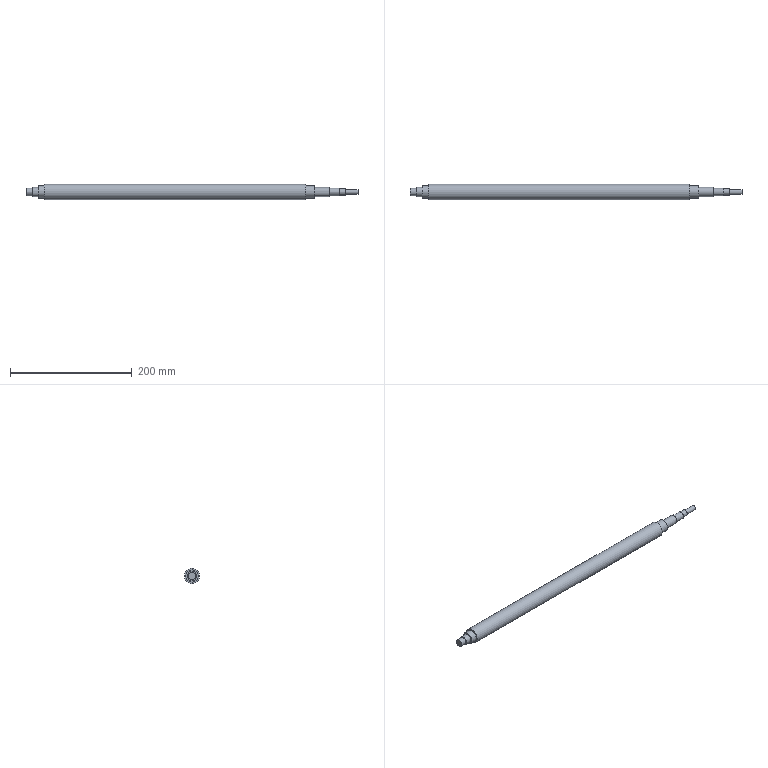Component | NX | X_LEADSCREW | 1 solid | 19 faces | box 546 x 25 x 25 mm | volume 229782 mm3 | plane 10 | cylinder 9 | commonest cylinder face diameters 12 x2 15 x2 20 x2 8 x1 10 x1 25 x1
STEP:
#1=CARTESIAN_POINT('',(0.,0.,0.));
#2=DIRECTION('',(0.,0.,1.));
#3=DIRECTION('',(1.,0.,0.));
#4=AXIS2_PLACEMENT_3D('',#1,#2,#3);
#5=CARTESIAN_POINT('',(417.689,-150.302,-1579.));
#6=VERTEX_POINT('',#5);
#7=CARTESIAN_POINT('',(417.689,-150.302,-1573.));
#8=DIRECTION('',(1.,0.,0.));
#9=DIRECTION('',(0.,0.,-1.));
#10=AXIS2_PLACEMENT_3D('',#7,#8,#9);
#11=CIRCLE('',#10,6.);
#12=CARTESIAN_POINT('',(417.689,-150.302,-1573.));
#13=DIRECTION('',(1.,0.,0.));
#14=DIRECTION('',(0.,0.,-1.));
#15=AXIS2_PLACEMENT_3D('',#12,#13,#14);
#16=PLANE('',#15);
#17=CARTESIAN_POINT('',(0.,0.));
#18=DIRECTION('',(1.,0.));
#19=AXIS2_PLACEMENT_2D('',#17,#18);
#20=CIRCLE('',#19,6.);
#21=(GEOMETRIC_REPRESENTATION_CONTEXT(2)PARAMETRIC_REPRESENTATION_CONTEXT()REPRESENTATION_CONTEXT('',''));
#22=DEFINITIONAL_REPRESENTATION('',(#20),#21);
#23=PCURVE('',#16,#22);
#24=CARTESIAN_POINT('',(662.689,-150.302,-1573.));
#25=DIRECTION('',(1.,0.,0.));
#26=DIRECTION('',(0.,0.,-1.));
#27=AXIS2_PLACEMENT_3D('',#24,#25,#26);
#28=CYLINDRICAL_SURFACE('',#27,6.);
#29=CARTESIAN_POINT('',(0.,-245.));
#30=DIRECTION('',(1.,0.));
#31=VECTOR('',#30,1.);
#32=LINE('',#29,#31);
#33=(GEOMETRIC_REPRESENTATION_CONTEXT(2)PARAMETRIC_REPRESENTATION_CONTEXT()REPRESENTATION_CONTEXT('',''));
#34=DEFINITIONAL_REPRESENTATION('',(#32),#33);
#35=PCURVE('',#28,#34);
#36=SURFACE_CURVE('',#11,(#23,#35),.PCURVE_S1.);
#37=EDGE_CURVE('',#6,#6,#36,.T.);
#38=ORIENTED_EDGE('',*,*,#37,.F.);
#39=EDGE_LOOP('',(#38));
#40=FACE_BOUND('',#39,.T.);
#41=ADVANCED_FACE('',(#40),#16,.F.);
#42=CARTESIAN_POINT('',(963.689,-150.302,-1577.));
#43=VERTEX_POINT('',#42);
#44=CARTESIAN_POINT('',(963.689,-150.302,-1573.));
#45=DIRECTION('',(1.,0.,0.));
#46=DIRECTION('',(0.,0.,-1.));
#47=AXIS2_PLACEMENT_3D('',#44,#45,#46);
#48=CIRCLE('',#47,4.);
#49=CARTESIAN_POINT('',(963.689,-150.302,-1573.));
#50=DIRECTION('',(1.,0.,0.));
#51=DIRECTION('',(0.,0.,-1.));
#52=AXIS2_PLACEMENT_3D('',#49,#50,#51);
#53=PLANE('',#52);
#54=CARTESIAN_POINT('',(0.,0.));
#55=DIRECTION('',(1.,0.));
#56=AXIS2_PLACEMENT_2D('',#54,#55);
#57=CIRCLE('',#56,4.);
#58=(GEOMETRIC_REPRESENTATION_CONTEXT(2)PARAMETRIC_REPRESENTATION_CONTEXT()REPRESENTATION_CONTEXT('',''));
#59=DEFINITIONAL_REPRESENTATION('',(#57),#58);
#60=PCURVE('',#53,#59);
#61=CARTESIAN_POINT('',(662.689,-150.302,-1573.));
#62=DIRECTION('',(1.,0.,0.));
#63=DIRECTION('',(0.,0.,-1.));
#64=AXIS2_PLACEMENT_3D('',#61,#62,#63);
#65=CYLINDRICAL_SURFACE('',#64,4.);
#66=CARTESIAN_POINT('',(0.,301.));
#67=DIRECTION('',(1.,0.));
#68=VECTOR('',#67,1.);
#69=LINE('',#66,#68);
#70=(GEOMETRIC_REPRESENTATION_CONTEXT(2)PARAMETRIC_REPRESENTATION_CONTEXT()REPRESENTATION_CONTEXT('',''));
#71=DEFINITIONAL_REPRESENTATION('',(#69),#70);
#72=PCURVE('',#65,#71);
#73=SURFACE_CURVE('',#48,(#60,#72),.PCURVE_S1.);
#74=EDGE_CURVE('',#43,#43,#73,.T.);
#75=ORIENTED_EDGE('',*,*,#74,.T.);
#76=EDGE_LOOP('',(#75));
#77=FACE_BOUND('',#76,.T.);
#78=ADVANCED_FACE('',(#77),#53,.T.);
#79=ORIENTED_EDGE('',*,*,#74,.F.);
#80=CARTESIAN_POINT('',(943.689,-150.302,-1577.));
#81=VERTEX_POINT('',#80);
#82=CARTESIAN_POINT('',(943.689,-150.302,-1577.));
#83=CARTESIAN_POINT('',(963.689,-150.302,-1577.));
#84=B_SPLINE_CURVE_WITH_KNOTS('',1,(#82,#83),.UNSPECIFIED.,.F.,.F.,(2,2),(281.,301.),.PIECEWISE_BEZIER_KNOTS.);
#85=CARTESIAN_POINT('',(0.,0.));
#86=DIRECTION('',(0.,1.));
#87=VECTOR('',#86,1.);
#88=LINE('',#85,#87);
#89=(GEOMETRIC_REPRESENTATION_CONTEXT(2)PARAMETRIC_REPRESENTATION_CONTEXT()REPRESENTATION_CONTEXT('',''));
#90=DEFINITIONAL_REPRESENTATION('',(#88),#89);
#91=PCURVE('',#65,#90);
#92=CARTESIAN_POINT('',(6.283,0.));
#93=DIRECTION('',(0.,1.));
#94=VECTOR('',#93,1.);
#95=LINE('',#92,#94);
#96=(GEOMETRIC_REPRESENTATION_CONTEXT(2)PARAMETRIC_REPRESENTATION_CONTEXT()REPRESENTATION_CONTEXT('',''));
#97=DEFINITIONAL_REPRESENTATION('',(#95),#96);
#98=PCURVE('',#65,#97);
#99=SEAM_CURVE('',#84,(#91,#98),.PCURVE_S1.);
#100=EDGE_CURVE('',#81,#43,#99,.T.);
#101=ORIENTED_EDGE('',*,*,#100,.F.);
#102=CARTESIAN_POINT('',(943.689,-150.302,-1573.));
#103=DIRECTION('',(1.,0.,0.));
#104=DIRECTION('',(0.,0.,-1.));
#105=AXIS2_PLACEMENT_3D('',#102,#103,#104);
#106=CIRCLE('',#105,4.);
#107=CARTESIAN_POINT('',(0.,281.));
#108=DIRECTION('',(1.,0.));
#109=VECTOR('',#108,1.);
#110=LINE('',#107,#109);
#111=(GEOMETRIC_REPRESENTATION_CONTEXT(2)PARAMETRIC_REPRESENTATION_CONTEXT()REPRESENTATION_CONTEXT('',''));
#112=DEFINITIONAL_REPRESENTATION('',(#110),#111);
#113=PCURVE('',#65,#112);
#114=CARTESIAN_POINT('',(943.689,-150.302,-1568.));
#115=DIRECTION('',(-1.,0.,0.));
#116=DIRECTION('',(0.,0.,1.));
#117=AXIS2_PLACEMENT_3D('',#114,#115,#116);
#118=PLANE('',#117);
#119=CARTESIAN_POINT('',(-9.,0.));
#120=CARTESIAN_POINT('',(-9.,6.928));
#121=CARTESIAN_POINT('',(-3.,3.464));
#122=CARTESIAN_POINT('',(3.,0.));
#123=CARTESIAN_POINT('',(-3.,-3.464));
#124=CARTESIAN_POINT('',(-9.,-6.928));
#125=CARTESIAN_POINT('',(-9.,0.));
#126=(BOUNDED_CURVE()B_SPLINE_CURVE(2,(#119,#120,#121,#122,#123,#124,#125),.UNSPECIFIED.,.T.,.F.)B_SPLINE_CURVE_WITH_KNOTS((1,2,2,2,2,1),(-2.094,0.,2.094,4.189,6.283,8.378),.UNSPECIFIED.)CURVE()GEOMETRIC_REPRESENTATION_ITEM()RATIONAL_B_SPLINE_CURVE((1.,0.5,1.,0.5,1.,0.5,1.))REPRESENTATION_ITEM(''));
#127=(GEOMETRIC_REPRESENTATION_CONTEXT(2)PARAMETRIC_REPRESENTATION_CONTEXT()REPRESENTATION_CONTEXT('',''));
#128=DEFINITIONAL_REPRESENTATION('',(#126),#127);
#129=PCURVE('',#118,#128);
#130=SURFACE_CURVE('',#106,(#113,#129),.PCURVE_S1.);
#131=EDGE_CURVE('',#81,#81,#130,.T.);
#132=ORIENTED_EDGE('',*,*,#131,.T.);
#133=ORIENTED_EDGE('',*,*,#100,.T.);
#134=EDGE_LOOP('',(#79,#101,#132,#133));
#135=FACE_BOUND('',#134,.T.);
#136=ADVANCED_FACE('',(#135),#65,.T.);
#137=ORIENTED_EDGE('',*,*,#131,.F.);
#138=EDGE_LOOP('',(#137));
#139=FACE_BOUND('',#138,.T.);
#140=CARTESIAN_POINT('',(943.689,-150.302,-1578.));
#141=VERTEX_POINT('',#140);
#142=CARTESIAN_POINT('',(943.689,-150.302,-1573.));
#143=DIRECTION('',(1.,0.,0.));
#144=DIRECTION('',(0.,0.,-1.));
#145=AXIS2_PLACEMENT_3D('',#142,#143,#144);
#146=CIRCLE('',#145,5.);
#147=CARTESIAN_POINT('',(-10.,0.));
#148=CARTESIAN_POINT('',(-10.,8.66));
#149=CARTESIAN_POINT('',(-2.5,4.33));
#150=CARTESIAN_POINT('',(5.,0.));
#151=CARTESIAN_POINT('',(-2.5,-4.33));
#152=CARTESIAN_POINT('',(-10.,-8.66));
#153=CARTESIAN_POINT('',(-10.,0.));
#154=(BOUNDED_CURVE()B_SPLINE_CURVE(2,(#147,#148,#149,#150,#151,#152,#153),.UNSPECIFIED.,.T.,.F.)B_SPLINE_CURVE_WITH_KNOTS((1,2,2,2,2,1),(-2.094,0.,2.094,4.189,6.283,8.378),.UNSPECIFIED.)CURVE()GEOMETRIC_REPRESENTATION_ITEM()RATIONAL_B_SPLINE_CURVE((1.,0.5,1.,0.5,1.,0.5,1.))REPRESENTATION_ITEM(''));
#155=(GEOMETRIC_REPRESENTATION_CONTEXT(2)PARAMETRIC_REPRESENTATION_CONTEXT()REPRESENTATION_CONTEXT('',''));
#156=DEFINITIONAL_REPRESENTATION('',(#154),#155);
#157=PCURVE('',#118,#156);
#158=CARTESIAN_POINT('',(662.689,-150.302,-1573.));
#159=DIRECTION('',(1.,0.,0.));
#160=DIRECTION('',(0.,0.,-1.));
#161=AXIS2_PLACEMENT_3D('',#158,#159,#160);
#162=CYLINDRICAL_SURFACE('',#161,5.);
#163=CARTESIAN_POINT('',(0.,281.));
#164=DIRECTION('',(1.,0.));
#165=VECTOR('',#164,1.);
#166=LINE('',#163,#165);
#167=(GEOMETRIC_REPRESENTATION_CONTEXT(2)PARAMETRIC_REPRESENTATION_CONTEXT()REPRESENTATION_CONTEXT('',''));
#168=DEFINITIONAL_REPRESENTATION('',(#166),#167);
#169=PCURVE('',#162,#168);
#170=SURFACE_CURVE('',#146,(#157,#169),.PCURVE_S1.);
#171=EDGE_CURVE('',#141,#141,#170,.T.);
#172=ORIENTED_EDGE('',*,*,#171,.T.);
#173=EDGE_LOOP('',(#172));
#174=FACE_BOUND('',#173,.T.);
#175=ADVANCED_FACE('',(#139,#174),#118,.F.);
#176=ORIENTED_EDGE('',*,*,#171,.F.);
#177=CARTESIAN_POINT('',(933.689,-150.302,-1578.));
#178=VERTEX_POINT('',#177);
#179=CARTESIAN_POINT('',(933.689,-150.302,-1578.));
#180=CARTESIAN_POINT('',(943.689,-150.302,-1578.));
#181=B_SPLINE_CURVE_WITH_KNOTS('',1,(#179,#180),.UNSPECIFIED.,.F.,.F.,(2,2),(271.,281.),.PIECEWISE_BEZIER_KNOTS.);
#182=CARTESIAN_POINT('',(0.,0.));
#183=DIRECTION('',(0.,1.));
#184=VECTOR('',#183,1.);
#185=LINE('',#182,#184);
#186=(GEOMETRIC_REPRESENTATION_CONTEXT(2)PARAMETRIC_REPRESENTATION_CONTEXT()REPRESENTATION_CONTEXT('',''));
#187=DEFINITIONAL_REPRESENTATION('',(#185),#186);
#188=PCURVE('',#162,#187);
#189=CARTESIAN_POINT('',(6.283,0.));
#190=DIRECTION('',(0.,1.));
#191=VECTOR('',#190,1.);
#192=LINE('',#189,#191);
#193=(GEOMETRIC_REPRESENTATION_CONTEXT(2)PARAMETRIC_REPRESENTATION_CONTEXT()REPRESENTATION_CONTEXT('',''));
#194=DEFINITIONAL_REPRESENTATION('',(#192),#193);
#195=PCURVE('',#162,#194);
#196=SEAM_CURVE('',#181,(#188,#195),.PCURVE_S1.);
#197=EDGE_CURVE('',#178,#141,#196,.T.);
#198=ORIENTED_EDGE('',*,*,#197,.F.);
#199=CARTESIAN_POINT('',(933.689,-150.302,-1573.));
#200=DIRECTION('',(1.,0.,0.));
#201=DIRECTION('',(0.,0.,-1.));
#202=AXIS2_PLACEMENT_3D('',#199,#200,#201);
#203=CIRCLE('',#202,5.);
#204=CARTESIAN_POINT('',(0.,271.));
#205=DIRECTION('',(1.,0.));
#206=VECTOR('',#205,1.);
#207=LINE('',#204,#206);
#208=(GEOMETRIC_REPRESENTATION_CONTEXT(2)PARAMETRIC_REPRESENTATION_CONTEXT()REPRESENTATION_CONTEXT('',''));
#209=DEFINITIONAL_REPRESENTATION('',(#207),#208);
#210=PCURVE('',#162,#209);
#211=CARTESIAN_POINT('',(933.689,-150.302,-1567.));
#212=DIRECTION('',(-1.,0.,0.));
#213=DIRECTION('',(0.,0.,1.));
#214=AXIS2_PLACEMENT_3D('',#211,#212,#213);
#215=PLANE('',#214);
#216=CARTESIAN_POINT('',(-11.,0.));
#217=CARTESIAN_POINT('',(-11.,8.66));
#218=CARTESIAN_POINT('',(-3.5,4.33));
#219=CARTESIAN_POINT('',(4.,0.));
#220=CARTESIAN_POINT('',(-3.5,-4.33));
#221=CARTESIAN_POINT('',(-11.,-8.66));
#222=CARTESIAN_POINT('',(-11.,0.));
#223=(BOUNDED_CURVE()B_SPLINE_CURVE(2,(#216,#217,#218,#219,#220,#221,#222),.UNSPECIFIED.,.T.,.F.)B_SPLINE_CURVE_WITH_KNOTS((1,2,2,2,2,1),(-2.094,0.,2.094,4.189,6.283,8.378),.UNSPECIFIED.)CURVE()GEOMETRIC_REPRESENTATION_ITEM()RATIONAL_B_SPLINE_CURVE((1.,0.5,1.,0.5,1.,0.5,1.))REPRESENTATION_ITEM(''));
#224=(GEOMETRIC_REPRESENTATION_CONTEXT(2)PARAMETRIC_REPRESENTATION_CONTEXT()REPRESENTATION_CONTEXT('',''));
#225=DEFINITIONAL_REPRESENTATION('',(#223),#224);
#226=PCURVE('',#215,#225);
#227=SURFACE_CURVE('',#203,(#210,#226),.PCURVE_S1.);
#228=EDGE_CURVE('',#178,#178,#227,.T.);
#229=ORIENTED_EDGE('',*,*,#228,.T.);
#230=ORIENTED_EDGE('',*,*,#197,.T.);
#231=EDGE_LOOP('',(#176,#198,#229,#230));
#232=FACE_BOUND('',#231,.T.);
#233=ADVANCED_FACE('',(#232),#162,.T.);
#234=ORIENTED_EDGE('',*,*,#228,.F.);
#235=EDGE_LOOP('',(#234));
#236=FACE_BOUND('',#235,.T.);
#237=CARTESIAN_POINT('',(933.689,-150.302,-1579.));
#238=VERTEX_POINT('',#237);
#239=CARTESIAN_POINT('',(933.689,-150.302,-1573.));
#240=DIRECTION('',(1.,0.,0.));
#241=DIRECTION('',(0.,0.,-1.));
#242=AXIS2_PLACEMENT_3D('',#239,#240,#241);
#243=CIRCLE('',#242,6.);
#244=CARTESIAN_POINT('',(-12.,0.));
#245=CARTESIAN_POINT('',(-12.,10.392));
#246=CARTESIAN_POINT('',(-3.,5.196));
#247=CARTESIAN_POINT('',(6.,0.));
#248=CARTESIAN_POINT('',(-3.,-5.196));
#249=CARTESIAN_POINT('',(-12.,-10.392));
#250=CARTESIAN_POINT('',(-12.,0.));
#251=(BOUNDED_CURVE()B_SPLINE_CURVE(2,(#244,#245,#246,#247,#248,#249,#250),.UNSPECIFIED.,.T.,.F.)B_SPLINE_CURVE_WITH_KNOTS((1,2,2,2,2,1),(-2.094,0.,2.094,4.189,6.283,8.378),.UNSPECIFIED.)CURVE()GEOMETRIC_REPRESENTATION_ITEM()RATIONAL_B_SPLINE_CURVE((1.,0.5,1.,0.5,1.,0.5,1.))REPRESENTATION_ITEM(''));
#252=(GEOMETRIC_REPRESENTATION_CONTEXT(2)PARAMETRIC_REPRESENTATION_CONTEXT()REPRESENTATION_CONTEXT('',''));
#253=DEFINITIONAL_REPRESENTATION('',(#251),#252);
#254=PCURVE('',#215,#253);
#255=CARTESIAN_POINT('',(662.689,-150.302,-1573.));
#256=DIRECTION('',(1.,0.,0.));
#257=DIRECTION('',(0.,0.,-1.));
#258=AXIS2_PLACEMENT_3D('',#255,#256,#257);
#259=CYLINDRICAL_SURFACE('',#258,6.);
#260=CARTESIAN_POINT('',(0.,271.));
#261=DIRECTION('',(1.,0.));
#262=VECTOR('',#261,1.);
#263=LINE('',#260,#262);
#264=(GEOMETRIC_REPRESENTATION_CONTEXT(2)PARAMETRIC_REPRESENTATION_CONTEXT()REPRESENTATION_CONTEXT('',''));
#265=DEFINITIONAL_REPRESENTATION('',(#263),#264);
#266=PCURVE('',#259,#265);
#267=SURFACE_CURVE('',#243,(#254,#266),.PCURVE_S1.);
#268=EDGE_CURVE('',#238,#238,#267,.T.);
#269=ORIENTED_EDGE('',*,*,#268,.T.);
#270=EDGE_LOOP('',(#269));
#271=FACE_BOUND('',#270,.T.);
#272=ADVANCED_FACE('',(#236,#271),#215,.F.);
#273=ORIENTED_EDGE('',*,*,#268,.F.);
#274=CARTESIAN_POINT('',(916.689,-150.302,-1579.));
#275=VERTEX_POINT('',#274);
#276=CARTESIAN_POINT('',(916.689,-150.302,-1579.));
#277=CARTESIAN_POINT('',(933.689,-150.302,-1579.));
#278=B_SPLINE_CURVE_WITH_KNOTS('',1,(#276,#277),.UNSPECIFIED.,.F.,.F.,(2,2),(254.,271.),.PIECEWISE_BEZIER_KNOTS.);
#279=CARTESIAN_POINT('',(0.,0.));
#280=DIRECTION('',(0.,1.));
#281=VECTOR('',#280,1.);
#282=LINE('',#279,#281);
#283=(GEOMETRIC_REPRESENTATION_CONTEXT(2)PARAMETRIC_REPRESENTATION_CONTEXT()REPRESENTATION_CONTEXT('',''));
#284=DEFINITIONAL_REPRESENTATION('',(#282),#283);
#285=PCURVE('',#259,#284);
#286=CARTESIAN_POINT('',(6.283,0.));
#287=DIRECTION('',(0.,1.));
#288=VECTOR('',#287,1.);
#289=LINE('',#286,#288);
#290=(GEOMETRIC_REPRESENTATION_CONTEXT(2)PARAMETRIC_REPRESENTATION_CONTEXT()REPRESENTATION_CONTEXT('',''));
#291=DEFINITIONAL_REPRESENTATION('',(#289),#290);
#292=PCURVE('',#259,#291);
#293=SEAM_CURVE('',#278,(#285,#292),.PCURVE_S1.);
#294=EDGE_CURVE('',#275,#238,#293,.T.);
#295=ORIENTED_EDGE('',*,*,#294,.F.);
#296=CARTESIAN_POINT('',(916.689,-150.302,-1573.));
#297=DIRECTION('',(1.,0.,0.));
#298=DIRECTION('',(0.,0.,-1.));
#299=AXIS2_PLACEMENT_3D('',#296,#297,#298);
#300=CIRCLE('',#299,6.);
#301=CARTESIAN_POINT('',(0.,254.));
#302=DIRECTION('',(1.,0.));
#303=VECTOR('',#302,1.);
#304=LINE('',#301,#303);
#305=(GEOMETRIC_REPRESENTATION_CONTEXT(2)PARAMETRIC_REPRESENTATION_CONTEXT()REPRESENTATION_CONTEXT('',''));
#306=DEFINITIONAL_REPRESENTATION('',(#304),#305);
#307=PCURVE('',#259,#306);
#308=CARTESIAN_POINT('',(916.689,-150.302,-1565.5));
#309=DIRECTION('',(-1.,0.,0.));
#310=DIRECTION('',(0.,0.,1.));
#311=AXIS2_PLACEMENT_3D('',#308,#309,#310);
#312=PLANE('',#311);
#313=CARTESIAN_POINT('',(-13.5,0.));
#314=CARTESIAN_POINT('',(-13.5,10.392));
#315=CARTESIAN_POINT('',(-4.5,5.196));
#316=CARTESIAN_POINT('',(4.5,0.));
#317=CARTESIAN_POINT('',(-4.5,-5.196));
#318=CARTESIAN_POINT('',(-13.5,-10.392));
#319=CARTESIAN_POINT('',(-13.5,0.));
#320=(BOUNDED_CURVE()B_SPLINE_CURVE(2,(#313,#314,#315,#316,#317,#318,#319),.UNSPECIFIED.,.T.,.F.)B_SPLINE_CURVE_WITH_KNOTS((1,2,2,2,2,1),(-2.094,0.,2.094,4.189,6.283,8.378),.UNSPECIFIED.)CURVE()GEOMETRIC_REPRESENTATION_ITEM()RATIONAL_B_SPLINE_CURVE((1.,0.5,1.,0.5,1.,0.5,1.))REPRESENTATION_ITEM(''));
#321=(GEOMETRIC_REPRESENTATION_CONTEXT(2)PARAMETRIC_REPRESENTATION_CONTEXT()REPRESENTATION_CONTEXT('',''));
#322=DEFINITIONAL_REPRESENTATION('',(#320),#321);
#323=PCURVE('',#312,#322);
#324=SURFACE_CURVE('',#300,(#307,#323),.PCURVE_S1.);
#325=EDGE_CURVE('',#275,#275,#324,.T.);
#326=ORIENTED_EDGE('',*,*,#325,.T.);
#327=ORIENTED_EDGE('',*,*,#294,.T.);
#328=EDGE_LOOP('',(#273,#295,#326,#327));
#329=FACE_BOUND('',#328,.T.);
#330=ADVANCED_FACE('',(#329),#259,.T.);
#331=ORIENTED_EDGE('',*,*,#325,.F.);
#332=EDGE_LOOP('',(#331));
#333=FACE_BOUND('',#332,.T.);
#334=CARTESIAN_POINT('',(916.689,-150.302,-1580.5));
#335=VERTEX_POINT('',#334);
#336=CARTESIAN_POINT('',(916.689,-150.302,-1573.));
#337=DIRECTION('',(1.,0.,0.));
#338=DIRECTION('',(0.,0.,-1.));
#339=AXIS2_PLACEMENT_3D('',#336,#337,#338);
#340=CIRCLE('',#339,7.5);
#341=CARTESIAN_POINT('',(-15.,0.));
#342=CARTESIAN_POINT('',(-15.,12.99));
#343=CARTESIAN_POINT('',(-3.75,6.495));
#344=CARTESIAN_POINT('',(7.5,0.));
#345=CARTESIAN_POINT('',(-3.75,-6.495));
#346=CARTESIAN_POINT('',(-15.,-12.99));
#347=CARTESIAN_POINT('',(-15.,0.));
#348=(BOUNDED_CURVE()B_SPLINE_CURVE(2,(#341,#342,#343,#344,#345,#346,#347),.UNSPECIFIED.,.T.,.F.)B_SPLINE_CURVE_WITH_KNOTS((1,2,2,2,2,1),(-2.094,0.,2.094,4.189,6.283,8.378),.UNSPECIFIED.)CURVE()GEOMETRIC_REPRESENTATION_ITEM()RATIONAL_B_SPLINE_CURVE((1.,0.5,1.,0.5,1.,0.5,1.))REPRESENTATION_ITEM(''));
#349=(GEOMETRIC_REPRESENTATION_CONTEXT(2)PARAMETRIC_REPRESENTATION_CONTEXT()REPRESENTATION_CONTEXT('',''));
#350=DEFINITIONAL_REPRESENTATION('',(#348),#349);
#351=PCURVE('',#312,#350);
#352=CARTESIAN_POINT('',(662.689,-150.302,-1573.));
#353=DIRECTION('',(1.,0.,0.));
#354=DIRECTION('',(0.,0.,-1.));
#355=AXIS2_PLACEMENT_3D('',#352,#353,#354);
#356=CYLINDRICAL_SURFACE('',#355,7.5);
#357=CARTESIAN_POINT('',(0.,254.));
#358=DIRECTION('',(1.,0.));
#359=VECTOR('',#358,1.);
#360=LINE('',#357,#359);
#361=(GEOMETRIC_REPRESENTATION_CONTEXT(2)PARAMETRIC_REPRESENTATION_CONTEXT()REPRESENTATION_CONTEXT('',''));
#362=DEFINITIONAL_REPRESENTATION('',(#360),#361);
#363=PCURVE('',#356,#362);
#364=SURFACE_CURVE('',#340,(#351,#363),.PCURVE_S1.);
#365=EDGE_CURVE('',#335,#335,#364,.T.);
#366=ORIENTED_EDGE('',*,*,#365,.T.);
#367=EDGE_LOOP('',(#366));
#368=FACE_BOUND('',#367,.T.);
#369=ADVANCED_FACE('',(#333,#368),#312,.F.);
#370=ORIENTED_EDGE('',*,*,#365,.F.);
#371=CARTESIAN_POINT('',(892.689,-150.302,-1580.5));
#372=VERTEX_POINT('',#371);
#373=CARTESIAN_POINT('',(892.689,-150.302,-1580.5));
#374=CARTESIAN_POINT('',(916.689,-150.302,-1580.5));
#375=B_SPLINE_CURVE_WITH_KNOTS('',1,(#373,#374),.UNSPECIFIED.,.F.,.F.,(2,2),(230.,254.),.PIECEWISE_BEZIER_KNOTS.);
#376=CARTESIAN_POINT('',(0.,0.));
#377=DIRECTION('',(0.,1.));
#378=VECTOR('',#377,1.);
#379=LINE('',#376,#378);
#380=(GEOMETRIC_REPRESENTATION_CONTEXT(2)PARAMETRIC_REPRESENTATION_CONTEXT()REPRESENTATION_CONTEXT('',''));
#381=DEFINITIONAL_REPRESENTATION('',(#379),#380);
#382=PCURVE('',#356,#381);
#383=CARTESIAN_POINT('',(6.283,0.));
#384=DIRECTION('',(0.,1.));
#385=VECTOR('',#384,1.);
#386=LINE('',#383,#385);
#387=(GEOMETRIC_REPRESENTATION_CONTEXT(2)PARAMETRIC_REPRESENTATION_CONTEXT()REPRESENTATION_CONTEXT('',''));
#388=DEFINITIONAL_REPRESENTATION('',(#386),#387);
#389=PCURVE('',#356,#388);
#390=SEAM_CURVE('',#375,(#382,#389),.PCURVE_S1.);
#391=EDGE_CURVE('',#372,#335,#390,.T.);
#392=ORIENTED_EDGE('',*,*,#391,.F.);
#393=CARTESIAN_POINT('',(892.689,-150.302,-1573.));
#394=DIRECTION('',(1.,0.,0.));
#395=DIRECTION('',(0.,0.,-1.));
#396=AXIS2_PLACEMENT_3D('',#393,#394,#395);
#397=CIRCLE('',#396,7.5);
#398=CARTESIAN_POINT('',(0.,230.));
#399=DIRECTION('',(1.,0.));
#400=VECTOR('',#399,1.);
#401=LINE('',#398,#400);
#402=(GEOMETRIC_REPRESENTATION_CONTEXT(2)PARAMETRIC_REPRESENTATION_CONTEXT()REPRESENTATION_CONTEXT('',''));
#403=DEFINITIONAL_REPRESENTATION('',(#401),#402);
#404=PCURVE('',#356,#403);
#405=CARTESIAN_POINT('',(892.689,-150.302,-1563.));
#406=DIRECTION('',(-1.,0.,0.));
#407=DIRECTION('',(0.,0.,1.));
#408=AXIS2_PLACEMENT_3D('',#405,#406,#407);
#409=PLANE('',#408);
#410=CARTESIAN_POINT('',(-17.5,0.));
#411=CARTESIAN_POINT('',(-17.5,12.99));
#412=CARTESIAN_POINT('',(-6.25,6.495));
#413=CARTESIAN_POINT('',(5.,0.));
#414=CARTESIAN_POINT('',(-6.25,-6.495));
#415=CARTESIAN_POINT('',(-17.5,-12.99));
#416=CARTESIAN_POINT('',(-17.5,0.));
#417=(BOUNDED_CURVE()B_SPLINE_CURVE(2,(#410,#411,#412,#413,#414,#415,#416),.UNSPECIFIED.,.T.,.F.)B_SPLINE_CURVE_WITH_KNOTS((1,2,2,2,2,1),(-2.094,0.,2.094,4.189,6.283,8.378),.UNSPECIFIED.)CURVE()GEOMETRIC_REPRESENTATION_ITEM()RATIONAL_B_SPLINE_CURVE((1.,0.5,1.,0.5,1.,0.5,1.))REPRESENTATION_ITEM(''));
#418=(GEOMETRIC_REPRESENTATION_CONTEXT(2)PARAMETRIC_REPRESENTATION_CONTEXT()REPRESENTATION_CONTEXT('',''));
#419=DEFINITIONAL_REPRESENTATION('',(#417),#418);
#420=PCURVE('',#409,#419);
#421=SURFACE_CURVE('',#397,(#404,#420),.PCURVE_S1.);
#422=EDGE_CURVE('',#372,#372,#421,.T.);
#423=ORIENTED_EDGE('',*,*,#422,.T.);
#424=ORIENTED_EDGE('',*,*,#391,.T.);
#425=EDGE_LOOP('',(#370,#392,#423,#424));
#426=FACE_BOUND('',#425,.T.);
#427=ADVANCED_FACE('',(#426),#356,.T.);
#428=ORIENTED_EDGE('',*,*,#422,.F.);
#429=EDGE_LOOP('',(#428));
#430=FACE_BOUND('',#429,.T.);
#431=CARTESIAN_POINT('',(892.689,-150.302,-1583.));
#432=VERTEX_POINT('',#431);
#433=CARTESIAN_POINT('',(892.689,-150.302,-1573.));
#434=DIRECTION('',(1.,0.,0.));
#435=DIRECTION('',(0.,0.,-1.));
#436=AXIS2_PLACEMENT_3D('',#433,#434,#435);
#437=CIRCLE('',#436,10.);
#438=CARTESIAN_POINT('',(-20.,0.));
#439=CARTESIAN_POINT('',(-20.,17.321));
#440=CARTESIAN_POINT('',(-5.,8.66));
#441=CARTESIAN_POINT('',(10.,0.));
#442=CARTESIAN_POINT('',(-5.,-8.66));
#443=CARTESIAN_POINT('',(-20.,-17.321));
#444=CARTESIAN_POINT('',(-20.,0.));
#445=(BOUNDED_CURVE()B_SPLINE_CURVE(2,(#438,#439,#440,#441,#442,#443,#444),.UNSPECIFIED.,.T.,.F.)B_SPLINE_CURVE_WITH_KNOTS((1,2,2,2,2,1),(-2.094,0.,2.094,4.189,6.283,8.378),.UNSPECIFIED.)CURVE()GEOMETRIC_REPRESENTATION_ITEM()RATIONAL_B_SPLINE_CURVE((1.,0.5,1.,0.5,1.,0.5,1.))REPRESENTATION_ITEM(''));
#446=(GEOMETRIC_REPRESENTATION_CONTEXT(2)PARAMETRIC_REPRESENTATION_CONTEXT()REPRESENTATION_CONTEXT('',''));
#447=DEFINITIONAL_REPRESENTATION('',(#445),#446);
#448=PCURVE('',#409,#447);
#449=CARTESIAN_POINT('',(662.689,-150.302,-1573.));
#450=DIRECTION('',(1.,0.,0.));
#451=DIRECTION('',(0.,0.,-1.));
#452=AXIS2_PLACEMENT_3D('',#449,#450,#451);
#453=CYLINDRICAL_SURFACE('',#452,10.);
#454=CARTESIAN_POINT('',(0.,230.));
#455=DIRECTION('',(1.,0.));
#456=VECTOR('',#455,1.);
#457=LINE('',#454,#456);
#458=(GEOMETRIC_REPRESENTATION_CONTEXT(2)PARAMETRIC_REPRESENTATION_CONTEXT()REPRESENTATION_CONTEXT('',''));
#459=DEFINITIONAL_REPRESENTATION('',(#457),#458);
#460=PCURVE('',#453,#459);
#461=SURFACE_CURVE('',#437,(#448,#460),.PCURVE_S1.);
#462=EDGE_CURVE('',#432,#432,#461,.T.);
#463=ORIENTED_EDGE('',*,*,#462,.T.);
#464=EDGE_LOOP('',(#463));
#465=FACE_BOUND('',#464,.T.);
#466=ADVANCED_FACE('',(#430,#465),#409,.F.);
#467=ORIENTED_EDGE('',*,*,#462,.F.);
#468=CARTESIAN_POINT('',(877.689,-150.302,-1583.));
#469=VERTEX_POINT('',#468);
#470=CARTESIAN_POINT('',(877.689,-150.302,-1583.));
#471=CARTESIAN_POINT('',(892.689,-150.302,-1583.));
#472=B_SPLINE_CURVE_WITH_KNOTS('',1,(#470,#471),.UNSPECIFIED.,.F.,.F.,(2,2),(215.,230.),.PIECEWISE_BEZIER_KNOTS.);
#473=CARTESIAN_POINT('',(0.,0.));
#474=DIRECTION('',(0.,1.));
#475=VECTOR('',#474,1.);
#476=LINE('',#473,#475);
#477=(GEOMETRIC_REPRESENTATION_CONTEXT(2)PARAMETRIC_REPRESENTATION_CONTEXT()REPRESENTATION_CONTEXT('',''));
#478=DEFINITIONAL_REPRESENTATION('',(#476),#477);
#479=PCURVE('',#453,#478);
#480=CARTESIAN_POINT('',(6.283,0.));
#481=DIRECTION('',(0.,1.));
#482=VECTOR('',#481,1.);
#483=LINE('',#480,#482);
#484=(GEOMETRIC_REPRESENTATION_CONTEXT(2)PARAMETRIC_REPRESENTATION_CONTEXT()REPRESENTATION_CONTEXT('',''));
#485=DEFINITIONAL_REPRESENTATION('',(#483),#484);
#486=PCURVE('',#453,#485);
#487=SEAM_CURVE('',#472,(#479,#486),.PCURVE_S1.);
#488=EDGE_CURVE('',#469,#432,#487,.T.);
#489=ORIENTED_EDGE('',*,*,#488,.F.);
#490=CARTESIAN_POINT('',(877.689,-150.302,-1573.));
#491=DIRECTION('',(1.,0.,0.));
#492=DIRECTION('',(0.,0.,-1.));
#493=AXIS2_PLACEMENT_3D('',#490,#491,#492);
#494=CIRCLE('',#493,10.);
#495=CARTESIAN_POINT('',(0.,215.));
#496=DIRECTION('',(1.,0.));
#497=VECTOR('',#496,1.);
#498=LINE('',#495,#497);
#499=(GEOMETRIC_REPRESENTATION_CONTEXT(2)PARAMETRIC_REPRESENTATION_CONTEXT()REPRESENTATION_CONTEXT('',''));
#500=DEFINITIONAL_REPRESENTATION('',(#498),#499);
#501=PCURVE('',#453,#500);
#502=CARTESIAN_POINT('',(877.689,-150.302,-1560.5));
#503=DIRECTION('',(-1.,0.,0.));
#504=DIRECTION('',(0.,0.,1.));
#505=AXIS2_PLACEMENT_3D('',#502,#503,#504);
#506=PLANE('',#505);
#507=CARTESIAN_POINT('',(-22.5,0.));
#508=CARTESIAN_POINT('',(-22.5,17.321));
#509=CARTESIAN_POINT('',(-7.5,8.66));
#510=CARTESIAN_POINT('',(7.5,0.));
#511=CARTESIAN_POINT('',(-7.5,-8.66));
#512=CARTESIAN_POINT('',(-22.5,-17.321));
#513=CARTESIAN_POINT('',(-22.5,0.));
#514=(BOUNDED_CURVE()B_SPLINE_CURVE(2,(#507,#508,#509,#510,#511,#512,#513),.UNSPECIFIED.,.T.,.F.)B_SPLINE_CURVE_WITH_KNOTS((1,2,2,2,2,1),(-2.094,0.,2.094,4.189,6.283,8.378),.UNSPECIFIED.)CURVE()GEOMETRIC_REPRESENTATION_ITEM()RATIONAL_B_SPLINE_CURVE((1.,0.5,1.,0.5,1.,0.5,1.))REPRESENTATION_ITEM(''));
#515=(GEOMETRIC_REPRESENTATION_CONTEXT(2)PARAMETRIC_REPRESENTATION_CONTEXT()REPRESENTATION_CONTEXT('',''));
#516=DEFINITIONAL_REPRESENTATION('',(#514),#515);
#517=PCURVE('',#506,#516);
#518=SURFACE_CURVE('',#494,(#501,#517),.PCURVE_S1.);
#519=EDGE_CURVE('',#469,#469,#518,.T.);
#520=ORIENTED_EDGE('',*,*,#519,.T.);
#521=ORIENTED_EDGE('',*,*,#488,.T.);
#522=EDGE_LOOP('',(#467,#489,#520,#521));
#523=FACE_BOUND('',#522,.T.);
#524=ADVANCED_FACE('',(#523),#453,.T.);
#525=ORIENTED_EDGE('',*,*,#519,.F.);
#526=EDGE_LOOP('',(#525));
#527=FACE_BOUND('',#526,.T.);
#528=CARTESIAN_POINT('',(877.689,-150.302,-1585.5));
#529=VERTEX_POINT('',#528);
#530=CARTESIAN_POINT('',(877.689,-150.302,-1573.));
#531=DIRECTION('',(1.,0.,0.));
#532=DIRECTION('',(0.,0.,-1.));
#533=AXIS2_PLACEMENT_3D('',#530,#531,#532);
#534=CIRCLE('',#533,12.5);
#535=CARTESIAN_POINT('',(-25.,0.));
#536=CARTESIAN_POINT('',(-25.,21.651));
#537=CARTESIAN_POINT('',(-6.25,10.825));
#538=CARTESIAN_POINT('',(12.5,0.));
#539=CARTESIAN_POINT('',(-6.25,-10.825));
#540=CARTESIAN_POINT('',(-25.,-21.651));
#541=CARTESIAN_POINT('',(-25.,0.));
#542=(BOUNDED_CURVE()B_SPLINE_CURVE(2,(#535,#536,#537,#538,#539,#540,#541),.UNSPECIFIED.,.T.,.F.)B_SPLINE_CURVE_WITH_KNOTS((1,2,2,2,2,1),(-2.094,0.,2.094,4.189,6.283,8.378),.UNSPECIFIED.)CURVE()GEOMETRIC_REPRESENTATION_ITEM()RATIONAL_B_SPLINE_CURVE((1.,0.5,1.,0.5,1.,0.5,1.))REPRESENTATION_ITEM(''));
#543=(GEOMETRIC_REPRESENTATION_CONTEXT(2)PARAMETRIC_REPRESENTATION_CONTEXT()REPRESENTATION_CONTEXT('',''));
#544=DEFINITIONAL_REPRESENTATION('',(#542),#543);
#545=PCURVE('',#506,#544);
#546=CARTESIAN_POINT('',(662.689,-150.302,-1573.));
#547=DIRECTION('',(1.,0.,0.));
#548=DIRECTION('',(0.,0.,-1.));
#549=AXIS2_PLACEMENT_3D('',#546,#547,#548);
#550=CYLINDRICAL_SURFACE('',#549,12.5);
#551=CARTESIAN_POINT('',(0.,215.));
#552=DIRECTION('',(1.,0.));
#553=VECTOR('',#552,1.);
#554=LINE('',#551,#553);
#555=(GEOMETRIC_REPRESENTATION_CONTEXT(2)PARAMETRIC_REPRESENTATION_CONTEXT()REPRESENTATION_CONTEXT('',''));
#556=DEFINITIONAL_REPRESENTATION('',(#554),#555);
#557=PCURVE('',#550,#556);
#558=SURFACE_CURVE('',#534,(#545,#557),.PCURVE_S1.);
#559=EDGE_CURVE('',#529,#529,#558,.T.);
#560=ORIENTED_EDGE('',*,*,#559,.T.);
#561=EDGE_LOOP('',(#560));
#562=FACE_BOUND('',#561,.T.);
#563=ADVANCED_FACE('',(#527,#562),#506,.F.);
#564=ORIENTED_EDGE('',*,*,#559,.F.);
#565=CARTESIAN_POINT('',(447.689,-150.302,-1585.5));
#566=VERTEX_POINT('',#565);
#567=CARTESIAN_POINT('',(447.689,-150.302,-1585.5));
#568=CARTESIAN_POINT('',(877.689,-150.302,-1585.5));
#569=B_SPLINE_CURVE_WITH_KNOTS('',1,(#567,#568),.UNSPECIFIED.,.F.,.F.,(2,2),(-215.,215.),.PIECEWISE_BEZIER_KNOTS.);
#570=CARTESIAN_POINT('',(0.,0.));
#571=DIRECTION('',(0.,1.));
#572=VECTOR('',#571,1.);
#573=LINE('',#570,#572);
#574=(GEOMETRIC_REPRESENTATION_CONTEXT(2)PARAMETRIC_REPRESENTATION_CONTEXT()REPRESENTATION_CONTEXT('',''));
#575=DEFINITIONAL_REPRESENTATION('',(#573),#574);
#576=PCURVE('',#550,#575);
#577=CARTESIAN_POINT('',(6.283,0.));
#578=DIRECTION('',(0.,1.));
#579=VECTOR('',#578,1.);
#580=LINE('',#577,#579);
#581=(GEOMETRIC_REPRESENTATION_CONTEXT(2)PARAMETRIC_REPRESENTATION_CONTEXT()REPRESENTATION_CONTEXT('',''));
#582=DEFINITIONAL_REPRESENTATION('',(#580),#581);
#583=PCURVE('',#550,#582);
#584=SEAM_CURVE('',#569,(#576,#583),.PCURVE_S1.);
#585=EDGE_CURVE('',#566,#529,#584,.T.);
#586=ORIENTED_EDGE('',*,*,#585,.F.);
#587=CARTESIAN_POINT('',(447.689,-150.302,-1573.));
#588=DIRECTION('',(1.,0.,0.));
#589=DIRECTION('',(0.,0.,-1.));
#590=AXIS2_PLACEMENT_3D('',#587,#588,#589);
#591=CIRCLE('',#590,12.5);
#592=CARTESIAN_POINT('',(0.,-215.));
#593=DIRECTION('',(1.,0.));
#594=VECTOR('',#593,1.);
#595=LINE('',#592,#594);
#596=(GEOMETRIC_REPRESENTATION_CONTEXT(2)PARAMETRIC_REPRESENTATION_CONTEXT()REPRESENTATION_CONTEXT('',''));
#597=DEFINITIONAL_REPRESENTATION('',(#595),#596);
#598=PCURVE('',#550,#597);
#599=CARTESIAN_POINT('',(447.689,-150.302,-1563.));
#600=DIRECTION('',(1.,0.,0.));
#601=DIRECTION('',(0.,0.,-1.));
#602=AXIS2_PLACEMENT_3D('',#599,#600,#601);
#603=PLANE('',#602);
#604=CARTESIAN_POINT('',(10.,0.));
#605=DIRECTION('',(1.,0.));
#606=AXIS2_PLACEMENT_2D('',#604,#605);
#607=CIRCLE('',#606,12.5);
#608=(GEOMETRIC_REPRESENTATION_CONTEXT(2)PARAMETRIC_REPRESENTATION_CONTEXT()REPRESENTATION_CONTEXT('',''));
#609=DEFINITIONAL_REPRESENTATION('',(#607),#608);
#610=PCURVE('',#603,#609);
#611=SURFACE_CURVE('',#591,(#598,#610),.PCURVE_S1.);
#612=EDGE_CURVE('',#566,#566,#611,.T.);
#613=ORIENTED_EDGE('',*,*,#612,.T.);
#614=ORIENTED_EDGE('',*,*,#585,.T.);
#615=EDGE_LOOP('',(#564,#586,#613,#614));
#616=FACE_BOUND('',#615,.T.);
#617=ADVANCED_FACE('',(#616),#550,.T.);
#618=ORIENTED_EDGE('',*,*,#612,.F.);
#619=EDGE_LOOP('',(#618));
#620=FACE_BOUND('',#619,.T.);
#621=CARTESIAN_POINT('',(447.689,-150.302,-1583.));
#622=VERTEX_POINT('',#621);
#623=CARTESIAN_POINT('',(447.689,-150.302,-1573.));
#624=DIRECTION('',(1.,0.,0.));
#625=DIRECTION('',(0.,0.,-1.));
#626=AXIS2_PLACEMENT_3D('',#623,#624,#625);
#627=CIRCLE('',#626,10.);
#628=CARTESIAN_POINT('',(10.,0.));
#629=DIRECTION('',(1.,0.));
#630=AXIS2_PLACEMENT_2D('',#628,#629);
#631=CIRCLE('',#630,10.);
#632=(GEOMETRIC_REPRESENTATION_CONTEXT(2)PARAMETRIC_REPRESENTATION_CONTEXT()REPRESENTATION_CONTEXT('',''));
#633=DEFINITIONAL_REPRESENTATION('',(#631),#632);
#634=PCURVE('',#603,#633);
#635=CARTESIAN_POINT('',(662.689,-150.302,-1573.));
#636=DIRECTION('',(1.,0.,0.));
#637=DIRECTION('',(0.,0.,-1.));
#638=AXIS2_PLACEMENT_3D('',#635,#636,#637);
#639=CYLINDRICAL_SURFACE('',#638,10.);
#640=CARTESIAN_POINT('',(0.,-215.));
#641=DIRECTION('',(1.,0.));
#642=VECTOR('',#641,1.);
#643=LINE('',#640,#642);
#644=(GEOMETRIC_REPRESENTATION_CONTEXT(2)PARAMETRIC_REPRESENTATION_CONTEXT()REPRESENTATION_CONTEXT('',''));
#645=DEFINITIONAL_REPRESENTATION('',(#643),#644);
#646=PCURVE('',#639,#645);
#647=SURFACE_CURVE('',#627,(#634,#646),.PCURVE_S1.);
#648=EDGE_CURVE('',#622,#622,#647,.T.);
#649=ORIENTED_EDGE('',*,*,#648,.T.);
#650=EDGE_LOOP('',(#649));
#651=FACE_BOUND('',#650,.T.);
#652=ADVANCED_FACE('',(#620,#651),#603,.F.);
#653=ORIENTED_EDGE('',*,*,#648,.F.);
#654=CARTESIAN_POINT('',(437.689,-150.302,-1583.));
#655=VERTEX_POINT('',#654);
#656=CARTESIAN_POINT('',(437.689,-150.302,-1583.));
#657=CARTESIAN_POINT('',(447.689,-150.302,-1583.));
#658=B_SPLINE_CURVE_WITH_KNOTS('',1,(#656,#657),.UNSPECIFIED.,.F.,.F.,(2,2),(-225.,-215.),.PIECEWISE_BEZIER_KNOTS.);
#659=CARTESIAN_POINT('',(0.,0.));
#660=DIRECTION('',(0.,1.));
#661=VECTOR('',#660,1.);
#662=LINE('',#659,#661);
#663=(GEOMETRIC_REPRESENTATION_CONTEXT(2)PARAMETRIC_REPRESENTATION_CONTEXT()REPRESENTATION_CONTEXT('',''));
#664=DEFINITIONAL_REPRESENTATION('',(#662),#663);
#665=PCURVE('',#639,#664);
#666=CARTESIAN_POINT('',(6.283,0.));
#667=DIRECTION('',(0.,1.));
#668=VECTOR('',#667,1.);
#669=LINE('',#666,#668);
#670=(GEOMETRIC_REPRESENTATION_CONTEXT(2)PARAMETRIC_REPRESENTATION_CONTEXT()REPRESENTATION_CONTEXT('',''));
#671=DEFINITIONAL_REPRESENTATION('',(#669),#670);
#672=PCURVE('',#639,#671);
#673=SEAM_CURVE('',#658,(#665,#672),.PCURVE_S1.);
#674=EDGE_CURVE('',#655,#622,#673,.T.);
#675=ORIENTED_EDGE('',*,*,#674,.F.);
#676=CARTESIAN_POINT('',(437.689,-150.302,-1573.));
#677=DIRECTION('',(1.,0.,0.));
#678=DIRECTION('',(0.,0.,-1.));
#679=AXIS2_PLACEMENT_3D('',#676,#677,#678);
#680=CIRCLE('',#679,10.);
#681=CARTESIAN_POINT('',(0.,-225.));
#682=DIRECTION('',(1.,0.));
#683=VECTOR('',#682,1.);
#684=LINE('',#681,#683);
#685=(GEOMETRIC_REPRESENTATION_CONTEXT(2)PARAMETRIC_REPRESENTATION_CONTEXT()REPRESENTATION_CONTEXT('',''));
#686=DEFINITIONAL_REPRESENTATION('',(#684),#685);
#687=PCURVE('',#639,#686);
#688=CARTESIAN_POINT('',(437.689,-150.302,-1565.5));
#689=DIRECTION('',(1.,0.,0.));
#690=DIRECTION('',(0.,0.,-1.));
#691=AXIS2_PLACEMENT_3D('',#688,#689,#690);
#692=PLANE('',#691);
#693=CARTESIAN_POINT('',(7.5,0.));
#694=DIRECTION('',(1.,0.));
#695=AXIS2_PLACEMENT_2D('',#693,#694);
#696=CIRCLE('',#695,10.);
#697=(GEOMETRIC_REPRESENTATION_CONTEXT(2)PARAMETRIC_REPRESENTATION_CONTEXT()REPRESENTATION_CONTEXT('',''));
#698=DEFINITIONAL_REPRESENTATION('',(#696),#697);
#699=PCURVE('',#692,#698);
#700=SURFACE_CURVE('',#680,(#687,#699),.PCURVE_S1.);
#701=EDGE_CURVE('',#655,#655,#700,.T.);
#702=ORIENTED_EDGE('',*,*,#701,.T.);
#703=ORIENTED_EDGE('',*,*,#674,.T.);
#704=EDGE_LOOP('',(#653,#675,#702,#703));
#705=FACE_BOUND('',#704,.T.);
#706=ADVANCED_FACE('',(#705),#639,.T.);
#707=ORIENTED_EDGE('',*,*,#701,.F.);
#708=EDGE_LOOP('',(#707));
#709=FACE_BOUND('',#708,.T.);
#710=CARTESIAN_POINT('',(437.689,-150.302,-1580.5));
#711=VERTEX_POINT('',#710);
#712=CARTESIAN_POINT('',(437.689,-150.302,-1573.));
#713=DIRECTION('',(1.,0.,0.));
#714=DIRECTION('',(0.,0.,-1.));
#715=AXIS2_PLACEMENT_3D('',#712,#713,#714);
#716=CIRCLE('',#715,7.5);
#717=CARTESIAN_POINT('',(7.5,0.));
#718=DIRECTION('',(1.,0.));
#719=AXIS2_PLACEMENT_2D('',#717,#718);
#720=CIRCLE('',#719,7.5);
#721=(GEOMETRIC_REPRESENTATION_CONTEXT(2)PARAMETRIC_REPRESENTATION_CONTEXT()REPRESENTATION_CONTEXT('',''));
#722=DEFINITIONAL_REPRESENTATION('',(#720),#721);
#723=PCURVE('',#692,#722);
#724=CARTESIAN_POINT('',(662.689,-150.302,-1573.));
#725=DIRECTION('',(1.,0.,0.));
#726=DIRECTION('',(0.,0.,-1.));
#727=AXIS2_PLACEMENT_3D('',#724,#725,#726);
#728=CYLINDRICAL_SURFACE('',#727,7.5);
#729=CARTESIAN_POINT('',(0.,-225.));
#730=DIRECTION('',(1.,0.));
#731=VECTOR('',#730,1.);
#732=LINE('',#729,#731);
#733=(GEOMETRIC_REPRESENTATION_CONTEXT(2)PARAMETRIC_REPRESENTATION_CONTEXT()REPRESENTATION_CONTEXT('',''));
#734=DEFINITIONAL_REPRESENTATION('',(#732),#733);
#735=PCURVE('',#728,#734);
#736=SURFACE_CURVE('',#716,(#723,#735),.PCURVE_S1.);
#737=EDGE_CURVE('',#711,#711,#736,.T.);
#738=ORIENTED_EDGE('',*,*,#737,.T.);
#739=EDGE_LOOP('',(#738));
#740=FACE_BOUND('',#739,.T.);
#741=ADVANCED_FACE('',(#709,#740),#692,.F.);
#742=ORIENTED_EDGE('',*,*,#737,.F.);
#743=CARTESIAN_POINT('',(427.689,-150.302,-1580.5));
#744=VERTEX_POINT('',#743);
#745=CARTESIAN_POINT('',(427.689,-150.302,-1580.5));
#746=CARTESIAN_POINT('',(437.689,-150.302,-1580.5));
#747=B_SPLINE_CURVE_WITH_KNOTS('',1,(#745,#746),.UNSPECIFIED.,.F.,.F.,(2,2),(-235.,-225.),.PIECEWISE_BEZIER_KNOTS.);
#748=CARTESIAN_POINT('',(0.,0.));
#749=DIRECTION('',(0.,1.));
#750=VECTOR('',#749,1.);
#751=LINE('',#748,#750);
#752=(GEOMETRIC_REPRESENTATION_CONTEXT(2)PARAMETRIC_REPRESENTATION_CONTEXT()REPRESENTATION_CONTEXT('',''));
#753=DEFINITIONAL_REPRESENTATION('',(#751),#752);
#754=PCURVE('',#728,#753);
#755=CARTESIAN_POINT('',(6.283,0.));
#756=DIRECTION('',(0.,1.));
#757=VECTOR('',#756,1.);
#758=LINE('',#755,#757);
#759=(GEOMETRIC_REPRESENTATION_CONTEXT(2)PARAMETRIC_REPRESENTATION_CONTEXT()REPRESENTATION_CONTEXT('',''));
#760=DEFINITIONAL_REPRESENTATION('',(#758),#759);
#761=PCURVE('',#728,#760);
#762=SEAM_CURVE('',#747,(#754,#761),.PCURVE_S1.);
#763=EDGE_CURVE('',#744,#711,#762,.T.);
#764=ORIENTED_EDGE('',*,*,#763,.F.);
#765=CARTESIAN_POINT('',(427.689,-150.302,-1573.));
#766=DIRECTION('',(1.,0.,0.));
#767=DIRECTION('',(0.,0.,-1.));
#768=AXIS2_PLACEMENT_3D('',#765,#766,#767);
#769=CIRCLE('',#768,7.5);
#770=CARTESIAN_POINT('',(0.,-235.));
#771=DIRECTION('',(1.,0.));
#772=VECTOR('',#771,1.);
#773=LINE('',#770,#772);
#774=(GEOMETRIC_REPRESENTATION_CONTEXT(2)PARAMETRIC_REPRESENTATION_CONTEXT()REPRESENTATION_CONTEXT('',''));
#775=DEFINITIONAL_REPRESENTATION('',(#773),#774);
#776=PCURVE('',#728,#775);
#777=CARTESIAN_POINT('',(427.689,-150.302,-1567.));
#778=DIRECTION('',(1.,0.,0.));
#779=DIRECTION('',(0.,0.,-1.));
#780=AXIS2_PLACEMENT_3D('',#777,#778,#779);
#781=PLANE('',#780);
#782=CARTESIAN_POINT('',(6.,0.));
#783=DIRECTION('',(1.,0.));
#784=AXIS2_PLACEMENT_2D('',#782,#783);
#785=CIRCLE('',#784,7.5);
#786=(GEOMETRIC_REPRESENTATION_CONTEXT(2)PARAMETRIC_REPRESENTATION_CONTEXT()REPRESENTATION_CONTEXT('',''));
#787=DEFINITIONAL_REPRESENTATION('',(#785),#786);
#788=PCURVE('',#781,#787);
#789=SURFACE_CURVE('',#769,(#776,#788),.PCURVE_S1.);
#790=EDGE_CURVE('',#744,#744,#789,.T.);
#791=ORIENTED_EDGE('',*,*,#790,.T.);
#792=ORIENTED_EDGE('',*,*,#763,.T.);
#793=EDGE_LOOP('',(#742,#764,#791,#792));
#794=FACE_BOUND('',#793,.T.);
#795=ADVANCED_FACE('',(#794),#728,.T.);
#796=ORIENTED_EDGE('',*,*,#790,.F.);
#797=EDGE_LOOP('',(#796));
#798=FACE_BOUND('',#797,.T.);
#799=CARTESIAN_POINT('',(427.689,-150.302,-1579.));
#800=VERTEX_POINT('',#799);
#801=CARTESIAN_POINT('',(427.689,-150.302,-1573.));
#802=DIRECTION('',(1.,0.,0.));
#803=DIRECTION('',(0.,0.,-1.));
#804=AXIS2_PLACEMENT_3D('',#801,#802,#803);
#805=CIRCLE('',#804,6.);
#806=CARTESIAN_POINT('',(6.,0.));
#807=DIRECTION('',(1.,0.));
#808=AXIS2_PLACEMENT_2D('',#806,#807);
#809=CIRCLE('',#808,6.);
#810=(GEOMETRIC_REPRESENTATION_CONTEXT(2)PARAMETRIC_REPRESENTATION_CONTEXT()REPRESENTATION_CONTEXT('',''));
#811=DEFINITIONAL_REPRESENTATION('',(#809),#810);
#812=PCURVE('',#781,#811);
#813=CARTESIAN_POINT('',(0.,-235.));
#814=DIRECTION('',(1.,0.));
#815=VECTOR('',#814,1.);
#816=LINE('',#813,#815);
#817=(GEOMETRIC_REPRESENTATION_CONTEXT(2)PARAMETRIC_REPRESENTATION_CONTEXT()REPRESENTATION_CONTEXT('',''));
#818=DEFINITIONAL_REPRESENTATION('',(#816),#817);
#819=PCURVE('',#28,#818);
#820=SURFACE_CURVE('',#805,(#812,#819),.PCURVE_S1.);
#821=EDGE_CURVE('',#800,#800,#820,.T.);
#822=ORIENTED_EDGE('',*,*,#821,.T.);
#823=EDGE_LOOP('',(#822));
#824=FACE_BOUND('',#823,.T.);
#825=ADVANCED_FACE('',(#798,#824),#781,.F.);
#826=ORIENTED_EDGE('',*,*,#821,.F.);
#827=CARTESIAN_POINT('',(417.689,-150.302,-1579.));
#828=CARTESIAN_POINT('',(427.689,-150.302,-1579.));
#829=B_SPLINE_CURVE_WITH_KNOTS('',1,(#827,#828),.UNSPECIFIED.,.F.,.F.,(2,2),(-245.,-235.),.PIECEWISE_BEZIER_KNOTS.);
#830=CARTESIAN_POINT('',(0.,0.));
#831=DIRECTION('',(0.,1.));
#832=VECTOR('',#831,1.);
#833=LINE('',#830,#832);
#834=(GEOMETRIC_REPRESENTATION_CONTEXT(2)PARAMETRIC_REPRESENTATION_CONTEXT()REPRESENTATION_CONTEXT('',''));
#835=DEFINITIONAL_REPRESENTATION('',(#833),#834);
#836=PCURVE('',#28,#835);
#837=CARTESIAN_POINT('',(6.283,0.));
#838=DIRECTION('',(0.,1.));
#839=VECTOR('',#838,1.);
#840=LINE('',#837,#839);
#841=(GEOMETRIC_REPRESENTATION_CONTEXT(2)PARAMETRIC_REPRESENTATION_CONTEXT()REPRESENTATION_CONTEXT('',''));
#842=DEFINITIONAL_REPRESENTATION('',(#840),#841);
#843=PCURVE('',#28,#842);
#844=SEAM_CURVE('',#829,(#836,#843),.PCURVE_S1.);
#845=EDGE_CURVE('',#6,#800,#844,.T.);
#846=ORIENTED_EDGE('',*,*,#845,.F.);
#847=ORIENTED_EDGE('',*,*,#37,.T.);
#848=ORIENTED_EDGE('',*,*,#845,.T.);
#849=EDGE_LOOP('',(#826,#846,#847,#848));
#850=FACE_BOUND('',#849,.T.);
#851=ADVANCED_FACE('',(#850),#28,.T.);
#852=CLOSED_SHELL('',(#41,#78,#136,#175,#233,#272,#330,#369,#427,#466,#524,#563,#617,#652,#706,#741,#795,#825,#851));
#853=MANIFOLD_SOLID_BREP('',#852);
#854=(LENGTH_UNIT()NAMED_UNIT(*)SI_UNIT(.MILLI.,.METRE.));
#855=UNCERTAINTY_MEASURE_WITH_UNIT(LENGTH_MEASURE(0.00001),#854,'','');
#856=(NAMED_UNIT(*)PLANE_ANGLE_UNIT()SI_UNIT($,.RADIAN.));
#857=(NAMED_UNIT(*)SI_UNIT($,.STERADIAN.)SOLID_ANGLE_UNIT());
#858=(GEOMETRIC_REPRESENTATION_CONTEXT(3)GLOBAL_UNCERTAINTY_ASSIGNED_CONTEXT((#855))GLOBAL_UNIT_ASSIGNED_CONTEXT((#854,#856,#857))REPRESENTATION_CONTEXT('',''));
#859=ADVANCED_BREP_SHAPE_REPRESENTATION('',(#4,#853),#858);